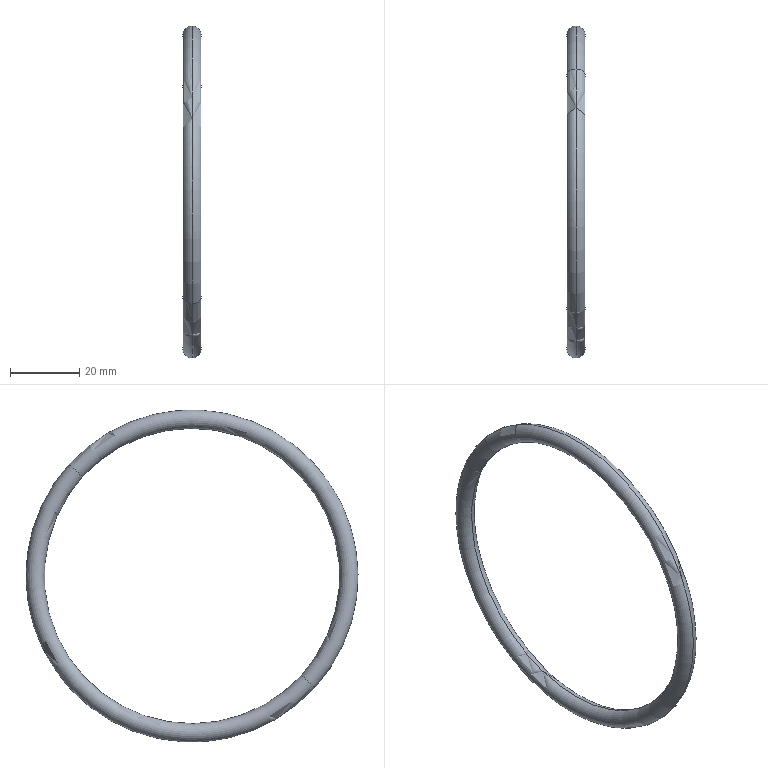Component | SolidWorks | SpringClipRubberRing-2 | 1 solid | 4 faces | box 5.3 x 95.7 x 95.7 mm | volume 6265 mm3 | torus 4 | material Silicone Rubber
build123d program:
from build123d import *

# Parameters (mm, degrees)
SKETCH1_R = 2.65


with BuildPart() as part:
    # Sketch1 → Revolve1 (revolve)
    with BuildSketch(Plane.XY, mode=Mode.PRIVATE) as revolve1_sk:
        with Locations((0, 45.199)):
            Circle(SKETCH1_R)
    revolve(revolve1_sk.sketch.rotate(Axis((0, 0, 0), (1, 0, 0)), 90), axis=Axis((0, 0, 0), (1, 0, 0)))


solid = part.part

# Placed as in the assembly
solid = solid.moved(Location((486.543, 0, 0), (0, 0, 0)))
STEP:
#1=COLOUR_RGB('',0.7922,0.8196,0.9333);
#2=FILL_AREA_STYLE_COLOUR('',#1);
#3=FILL_AREA_STYLE('',(#2));
#4=SURFACE_STYLE_FILL_AREA(#3);
#5=SURFACE_SIDE_STYLE('',(#4));
#6=SURFACE_STYLE_USAGE(.BOTH.,#5);
#7=PRESENTATION_STYLE_ASSIGNMENT((#6));
#8=CARTESIAN_POINT('',(19.155,-1.394,-1.267));
#9=VERTEX_POINT('',#8);
#10=CARTESIAN_POINT('',(19.155,-1.24,-1.127));
#11=VERTEX_POINT('',#10);
#12=CARTESIAN_POINT('',(19.155,-1.317,-1.197));
#13=DIRECTION('',(0.,0.6726,-0.74));
#14=DIRECTION('',(0.,0.74,0.6726));
#15=AXIS2_PLACEMENT_3D('',#12,#13,#14);
#16=CIRCLE('',#15,0.1043);
#17=EDGE_CURVE('',#9,#11,#16,.T.);
#18=ORIENTED_EDGE('',*,*,#17,.F.);
#19=CARTESIAN_POINT('',(19.155,1.394,1.267));
#20=VERTEX_POINT('',#19);
#21=CARTESIAN_POINT('',(19.155,-0.,0.));
#22=DIRECTION('',(-1.,0.,0.));
#23=DIRECTION('',(0.,0.,1.));
#24=AXIS2_PLACEMENT_3D('',#21,#22,#23);
#25=CIRCLE('',#24,1.884);
#26=EDGE_CURVE('',#9,#20,#25,.T.);
#27=ORIENTED_EDGE('',*,*,#26,.T.);
#28=CARTESIAN_POINT('',(19.155,1.24,1.127));
#29=VERTEX_POINT('',#28);
#30=CARTESIAN_POINT('',(19.155,1.317,1.197));
#31=DIRECTION('',(0.,-0.6726,0.74));
#32=DIRECTION('',(0.,-0.74,-0.6726));
#33=AXIS2_PLACEMENT_3D('',#30,#31,#32);
#34=CIRCLE('',#33,0.1043);
#35=EDGE_CURVE('',#20,#29,#34,.T.);
#36=ORIENTED_EDGE('',*,*,#35,.T.);
#37=CARTESIAN_POINT('',(19.155,-0.,0.));
#38=DIRECTION('',(-1.,0.,0.));
#39=DIRECTION('',(0.,0.,1.));
#40=AXIS2_PLACEMENT_3D('',#37,#38,#39);
#41=CIRCLE('',#40,1.675);
#42=EDGE_CURVE('',#11,#29,#41,.T.);
#43=ORIENTED_EDGE('',*,*,#42,.F.);
#44=EDGE_LOOP('',(#18,#27,#36,#43));
#45=FACE_OUTER_BOUND('',#44,.T.);
#46=CARTESIAN_POINT('',(19.155,-0.,0.));
#47=DIRECTION('',(-1.,0.,0.));
#48=DIRECTION('',(0.,0.74,0.6726));
#49=AXIS2_PLACEMENT_3D('',#46,#47,#48);
#50=TOROIDAL_SURFACE('',#49,1.779,0.1043);
#51=ADVANCED_FACE('',(#45),#50,.T.);
#52=ORIENTED_EDGE('',*,*,#35,.F.);
#53=CARTESIAN_POINT('',(19.155,-0.,0.));
#54=DIRECTION('',(-1.,0.,0.));
#55=DIRECTION('',(0.,0.,1.));
#56=AXIS2_PLACEMENT_3D('',#53,#54,#55);
#57=CIRCLE('',#56,1.884);
#58=EDGE_CURVE('',#20,#9,#57,.T.);
#59=ORIENTED_EDGE('',*,*,#58,.T.);
#60=ORIENTED_EDGE('',*,*,#17,.T.);
#61=CARTESIAN_POINT('',(19.155,-0.,0.));
#62=DIRECTION('',(-1.,0.,0.));
#63=DIRECTION('',(0.,0.,1.));
#64=AXIS2_PLACEMENT_3D('',#61,#62,#63);
#65=CIRCLE('',#64,1.675);
#66=EDGE_CURVE('',#29,#11,#65,.T.);
#67=ORIENTED_EDGE('',*,*,#66,.F.);
#68=EDGE_LOOP('',(#52,#59,#60,#67));
#69=FACE_OUTER_BOUND('',#68,.T.);
#70=CARTESIAN_POINT('',(19.155,-0.,0.));
#71=DIRECTION('',(-1.,0.,0.));
#72=DIRECTION('',(0.,0.74,0.6726));
#73=AXIS2_PLACEMENT_3D('',#70,#71,#72);
#74=TOROIDAL_SURFACE('',#73,1.779,0.1043);
#75=ADVANCED_FACE('',(#69),#74,.T.);
#76=ORIENTED_EDGE('',*,*,#58,.F.);
#77=CARTESIAN_POINT('',(19.155,1.317,1.197));
#78=DIRECTION('',(0.,-0.6726,0.74));
#79=DIRECTION('',(0.,-0.74,-0.6726));
#80=AXIS2_PLACEMENT_3D('',#77,#78,#79);
#81=CIRCLE('',#80,0.1043);
#82=EDGE_CURVE('',#29,#20,#81,.T.);
#83=ORIENTED_EDGE('',*,*,#82,.F.);
#84=ORIENTED_EDGE('',*,*,#66,.T.);
#85=CARTESIAN_POINT('',(19.155,-1.317,-1.197));
#86=DIRECTION('',(0.,0.6726,-0.74));
#87=DIRECTION('',(0.,0.74,0.6726));
#88=AXIS2_PLACEMENT_3D('',#85,#86,#87);
#89=CIRCLE('',#88,0.1043);
#90=EDGE_CURVE('',#11,#9,#89,.T.);
#91=ORIENTED_EDGE('',*,*,#90,.T.);
#92=EDGE_LOOP('',(#76,#83,#84,#91));
#93=FACE_OUTER_BOUND('',#92,.T.);
#94=CARTESIAN_POINT('',(19.155,-0.,0.));
#95=DIRECTION('',(-1.,0.,0.));
#96=DIRECTION('',(0.,0.74,0.6726));
#97=AXIS2_PLACEMENT_3D('',#94,#95,#96);
#98=TOROIDAL_SURFACE('',#97,1.779,0.1043);
#99=ADVANCED_FACE('',(#93),#98,.T.);
#100=ORIENTED_EDGE('',*,*,#26,.F.);
#101=ORIENTED_EDGE('',*,*,#90,.F.);
#102=ORIENTED_EDGE('',*,*,#42,.T.);
#103=ORIENTED_EDGE('',*,*,#82,.T.);
#104=EDGE_LOOP('',(#100,#101,#102,#103));
#105=FACE_OUTER_BOUND('',#104,.T.);
#106=CARTESIAN_POINT('',(19.155,-0.,0.));
#107=DIRECTION('',(-1.,0.,0.));
#108=DIRECTION('',(0.,0.74,0.6726));
#109=AXIS2_PLACEMENT_3D('',#106,#107,#108);
#110=TOROIDAL_SURFACE('',#109,1.779,0.1043);
#111=ADVANCED_FACE('',(#105),#110,.T.);
#112=CLOSED_SHELL('',(#51,#75,#99,#111));
#113=MANIFOLD_SOLID_BREP('',#112);
#114=STYLED_ITEM('',(#7),#113);
#115=(LENGTH_UNIT()NAMED_UNIT(*)SI_UNIT($,.METRE.));
#116=LENGTH_MEASURE_WITH_UNIT(LENGTH_MEASURE(0.0254),#115);
#117=DIMENSIONAL_EXPONENTS(1.,0.,0.,0.,0.,0.,0.);
#118=(CONVERSION_BASED_UNIT('',#116)LENGTH_UNIT()NAMED_UNIT(#117));
#119=UNCERTAINTY_MEASURE_WITH_UNIT(LENGTH_MEASURE(0.00001),#118,'','');
#120=(NAMED_UNIT(*)PLANE_ANGLE_UNIT()SI_UNIT($,.RADIAN.));
#121=(NAMED_UNIT(*)SI_UNIT($,.STERADIAN.)SOLID_ANGLE_UNIT());
#122=(GEOMETRIC_REPRESENTATION_CONTEXT(3)GLOBAL_UNCERTAINTY_ASSIGNED_CONTEXT((#119))GLOBAL_UNIT_ASSIGNED_CONTEXT((#118,#120,#121))REPRESENTATION_CONTEXT('',''));
#123=MECHANICAL_DESIGN_GEOMETRIC_PRESENTATION_REPRESENTATION('',(#114),#122);
#124=CARTESIAN_POINT('',(0.,0.,0.));
#125=DIRECTION('',(0.,0.,1.));
#126=DIRECTION('',(1.,0.,0.));
#127=AXIS2_PLACEMENT_3D('',#124,#125,#126);
#128=(LENGTH_UNIT()NAMED_UNIT(*)SI_UNIT($,.METRE.));
#129=LENGTH_MEASURE_WITH_UNIT(LENGTH_MEASURE(0.0254),#128);
#130=DIMENSIONAL_EXPONENTS(1.,0.,0.,0.,0.,0.,0.);
#131=(CONVERSION_BASED_UNIT('',#129)LENGTH_UNIT()NAMED_UNIT(#130));
#132=UNCERTAINTY_MEASURE_WITH_UNIT(LENGTH_MEASURE(0.00001),#131,'','');
#133=(NAMED_UNIT(*)PLANE_ANGLE_UNIT()SI_UNIT($,.RADIAN.));
#134=(NAMED_UNIT(*)SI_UNIT($,.STERADIAN.)SOLID_ANGLE_UNIT());
#135=(GEOMETRIC_REPRESENTATION_CONTEXT(3)GLOBAL_UNCERTAINTY_ASSIGNED_CONTEXT((#132))GLOBAL_UNIT_ASSIGNED_CONTEXT((#131,#133,#134))REPRESENTATION_CONTEXT('',''));
#136=ADVANCED_BREP_SHAPE_REPRESENTATION('',(#113,#127),#135);
#137=PRESENTATION_LAYER_ASSIGNMENT('','',(#114));